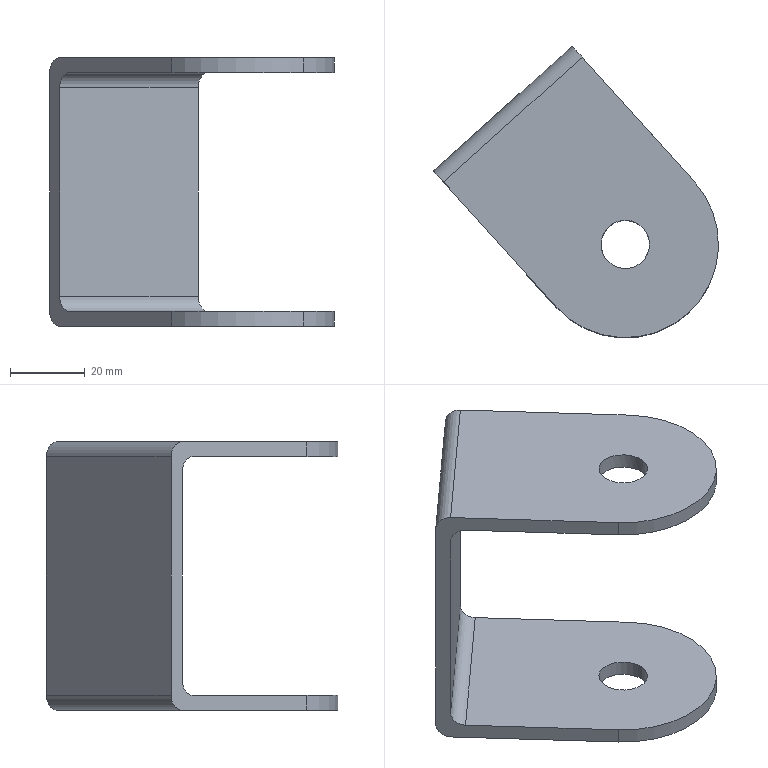Component | NX | ADJ_BRKT_CONN_LUG | 1 solid | 18 faces | volume 39192 mm3 | cylinder 10 | plane 8 | commonest cylinder face diameters 50 x4 8 x4 13 x2